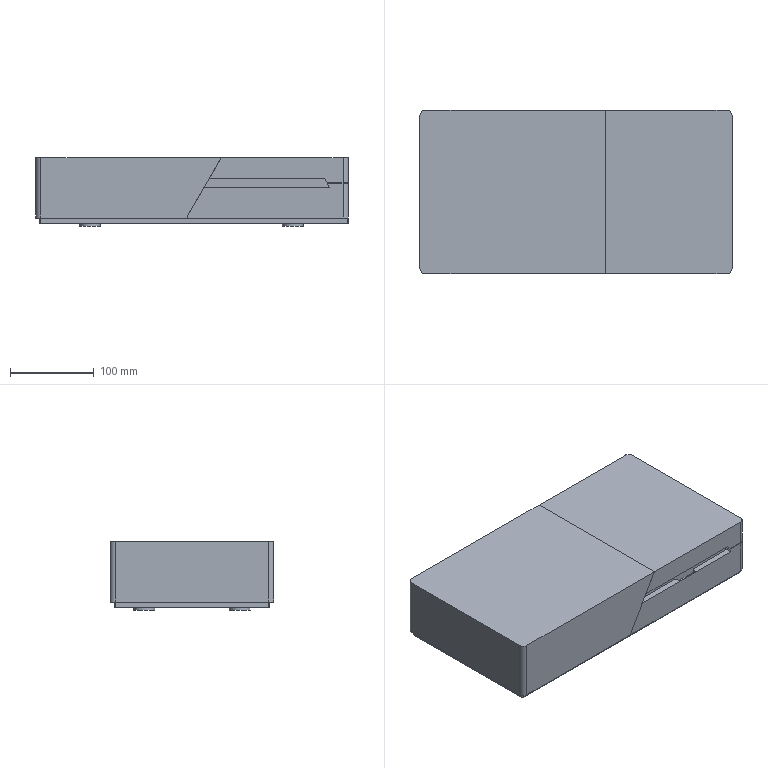Assembly | NX | mm | 12 component files | 16 solids | 526 faces | box 372 x 194.6 x 82 mm | volume 3248391 mm3 | plane 382 | cylinder 142 | torus 2 | commonest cylinder face diameters 1.5 x40 2.5 x16 1.2 x16 1 x16 2.8 x16 3 x14 12 x6 6 x6
Bill of materials:
unnamed part 1 | 1 |  | Open-top rectangular box with thin walls, split by internal partitions into three compartments: one long compartment along one side and two smaller compartments side by side.
unnamed part 2 | 2 |  | Long, narrow, thin strip or rail with a group of short and long rounded slots near one end and two small round features along its length; end view shows a thin profile with small stepped returns at both edges.
unnamed part 3 | 2 |  | Long, narrow, thin strip similar to a companion rail, with a group of rounded slots near one end and small round holes along its length; end view shows a thin profile with stepped returns at both edges.
unnamed part 4 | 1 |  | Shallow open tray with a flat floor and low side walls; one long wall is taller and runs past the tray, ending in an angled end at one side and a wider T-shaped end flange at the other. A rounded-edge notch is cut into the top of the taller wall.
unnamed part 5 | 1 |  | Cover-like part: a flat top plate with two downturned side walls forming an inverted U-channel, with one end cut at an angle and one rounded corner on the top plate.
unnamed part 6 | 1 |  | Shallow open tray with a flat floor and low walls, with a taller long wall that has an angled end and a T-shaped end flange; looks like a mirrored variant of the similar tray part, without an obvious notch in the tall wall.
unnamed part 7 | 1 |  | Rectangular open-top tray split by internal walls into several compartments of different sizes (about six), with a long rectangular slot through one long outer side wall near its base.
unnamed part 8 | 1 |  | Simple open-top rectangular box with thin walls and a single internal cavity, with no partitions.
unnamed part 9 | 1 |  | Thin rectangular plate with an upturned flange along one short edge and small round bosses or pins on both faces (two visible on top, two on the bottom).
unnamed part 10 | 1 |  | Solid rectangular slab or block with one end cut at an angle, rounded corners on the opposite end, and a small step on the underside near one end; top view shows a thin lip or flange along one edge.
Mates:
1. concentric | inner_box 1 edge | L_base 1 edge
2. concentric | inner_box 1 edge | L_base 1 edge
3. concentric | slide_rail_large 2 edge | inner_box 1 edge
4. concentric | slide_rail_large 2 edge | inner_box 1 edge
5. concentric | slide_rail_small 2 edge | inner_box 1 edge
6. concentric | slide_rail_small 2 edge | inner_box 1 edge
7. concentric | slide_rail_large 1 edge | inner_box 1 edge
8. concentric | slide_rail_large 1 edge | inner_box 1 edge
9. concentric | slide_rail_small 1 edge | inner_box 1 edge
10. concentric | slide_rail_small 1 edge | inner_box 1 edge
11. touch align | slide_cover_large 1 face | slide_rail_large 2 face
12. touch align | slide_cover_large 1 face | slide_rail_large 1 face
13. distance | slide_cover_large 1 face | inner_box 1 face
14. touch align | slide_cover_small 1 face | slide_rail_small 1 face
15. touch align | slide_cover_small 1 face | slide_rail_small 2 face
16. distance | inner_box 1 face | slide_cover_small 1 face
17. touch align | inner_box 1 face | drawer 1 face
18. distance | drawer 1 face | inner_box 1 face
19. parallel | drawer_2 1 face | inner_box 1 face
20. parallel | drawer_2 1 face | inner_box 1 face
21. distance | drawer_2 1 face | inner_box 1 face
22. distance | drawer_2 1 face | inner_box 1 face